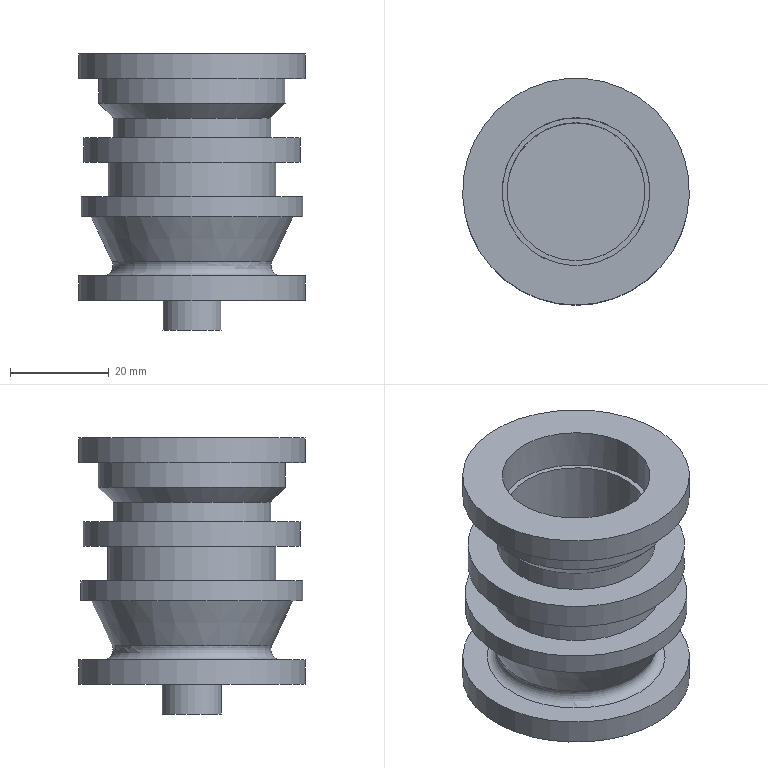Component | NX | LAMP_BODY | 1 solid | 24 faces | volume 31253 mm3 | plane 11 | cylinder 10 | cone 2 | torus 1 | commonest cylinder face diameters 46 x2 38 x1 32 x1 44 x1 34 x1 45 x1 12 x1 30 x1